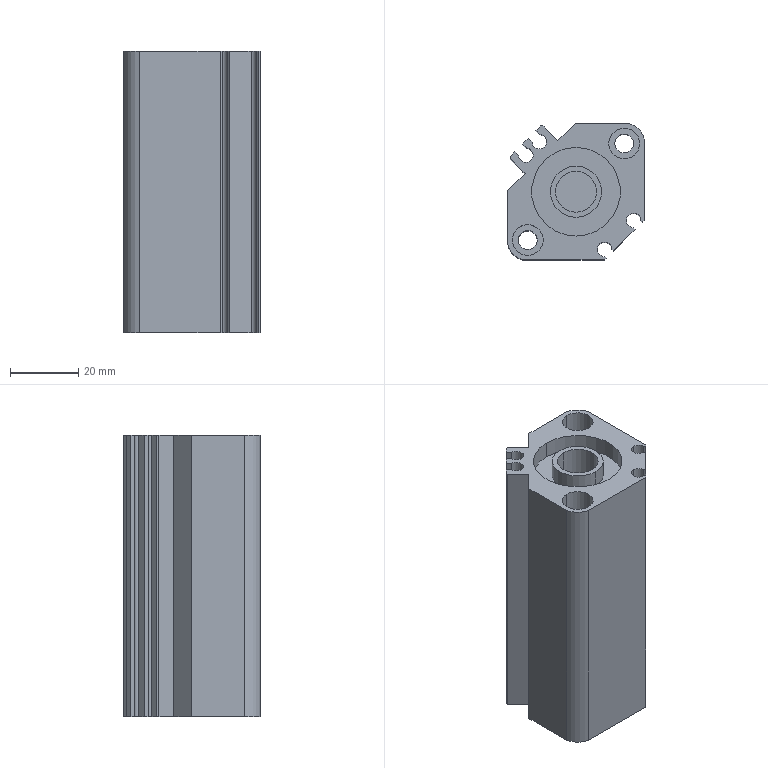Component | SolidWorks | CDQ2B25-50DZ-M9N(0_0_0)-1_CDQ2B25-50-M9N(0_0)_BODY-1 | 1 solid | 79 faces | volume 75142 mm3 | cylinder 38 | plane 37 | cone 4 | commonest cylinder face diameters 4.26 x10 9 x8 5.5 x4 4.134 x4 12 x4 26 x4 25 x2 15 x2